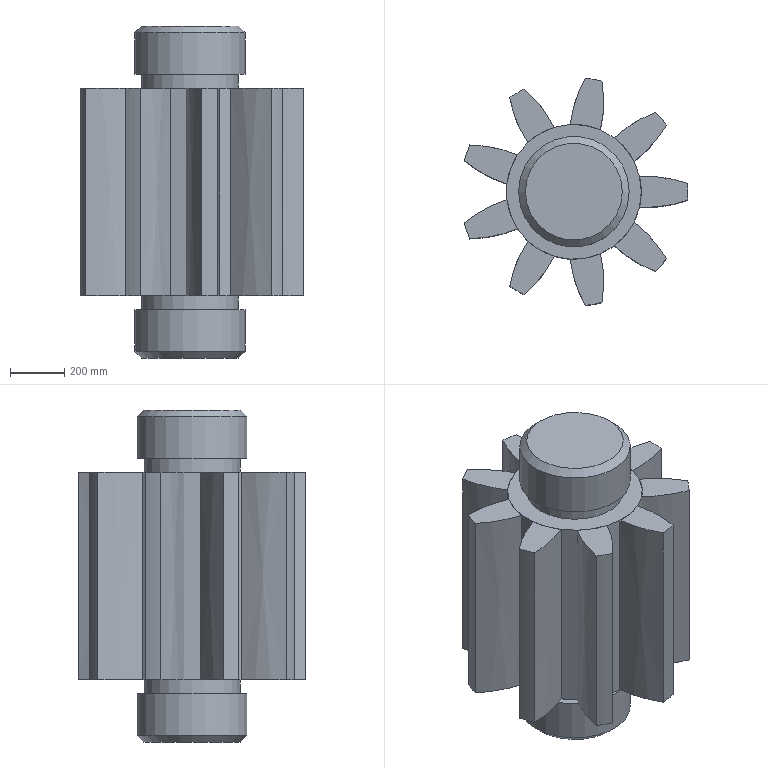Component | NX | 2 | 10 solids | 67 faces | volume 319213082 mm3 | plane 24 | cylinder 23 | other 18 | cone 2 | commonest cylinder face diameters 495.3 x10 838.2 x9 355.6 x2 406.4 x2